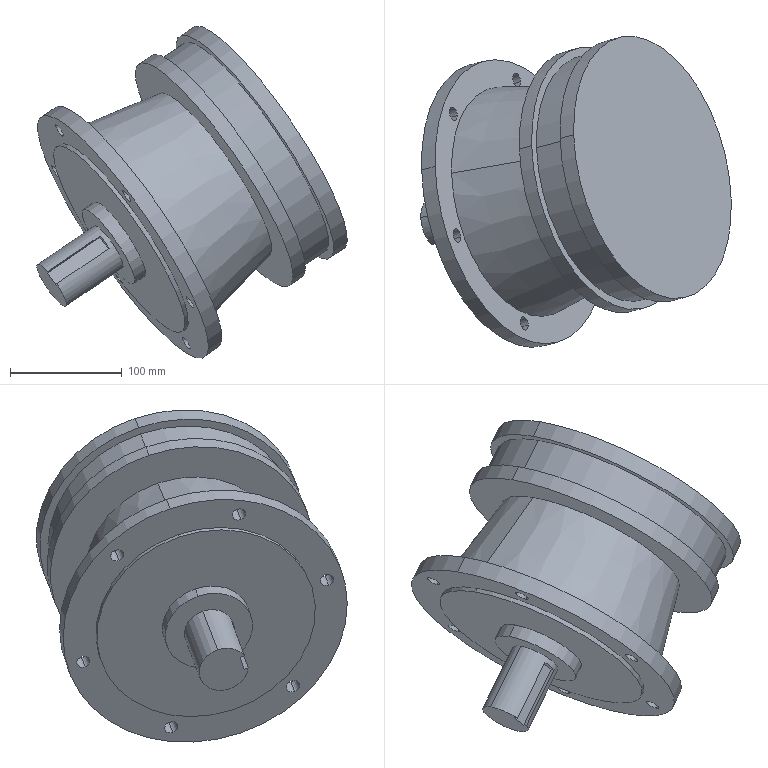Component | SolidWorks | XLD-4CycloidReducer-1 | 1 solid | 41 faces | box 277.92 x 278.17 x 297.34 mm | volume 6129226 mm3 | cylinder 26 | plane 13 | cone 2 | commonest cylinder face diameters 12.084 x12 240 x4 45 x2 80 x2 200 x2 260 x2 225.374 x2
build123d program:
from build123d import *

# Parameters (mm, degrees)
SKETCH2_R          = 40
EXTRUDE1_DEPTH     = 12
SKETCH3_R          = 22.5
EXTRUDE2_DEPTH     = 63
SKETCH4_W          = 14
SKETCH4_H          = 12.067
CUT_EXTRUDE1_DEPTH = 58
SKETCH5_R          = 6.042
CUT_EXTRUDE2_DEPTH = 40
CIRPATTERN1_COUNT  = 6


with BuildPart() as part:
    # Sketch1 → Revolve1 (revolve)
    with BuildSketch(Plane.XY, mode=Mode.PRIVATE) as revolve1_sk:
        Polygon((0, 0), (0, 100), (4, 100), (4, 130), (19, 130), (19, 105), (105, 87.671), (105, 120), (118.547, 120), (118.547, 112.687), (149.924, 112.687), (149.924, 120), (165, 120), (165, 0), align=None)
    revolve(revolve1_sk.sketch.rotate(Axis((0, 0, 0), (1, 0, 0)), 90), axis=Axis((0, 0, 0), (1, 0, 0)))

    # Sketch2 → Extrude1 (add)
    with BuildSketch(Plane.ZY):
        with Locations(Location((0, 0, 0), (0, 0, 180))):
            Circle(SKETCH2_R)
    extrude(amount=EXTRUDE1_DEPTH)

    # Sketch3 → Extrude2 (add)
    with BuildSketch(Plane.ZY.offset(12)):
        Circle(SKETCH3_R)
    extrude(amount=EXTRUDE2_DEPTH)

    # Sketch4 → Cut-Extrude1 (cut)
    with BuildSketch(Plane.ZY.offset(75)):
        with Locations((0, 23.534)):
            Rectangle(SKETCH4_W, SKETCH4_H)
    extrude(amount=-CUT_EXTRUDE1_DEPTH, mode=Mode.SUBTRACT)

    # Sketch5 → Cut-Extrude2 (cut)
    with BuildSketch(Plane.ZY.offset(-4)):
        with Locations((0, 115)):
            Circle(SKETCH5_R)
    cut_extrude2 = extrude(amount=-CUT_EXTRUDE2_DEPTH, mode=Mode.SUBTRACT)

    # CirPattern1: Cut-Extrude2 ×6 about axis
    cirpattern1_axis = Axis((0, 0, 0), (1, 0, 0))
    for i in range(1, CIRPATTERN1_COUNT):
        add(cut_extrude2.rotate(cirpattern1_axis, i * 360 / CIRPATTERN1_COUNT), mode=Mode.SUBTRACT)


solid = part.part

# Placed as in the assembly
solid = solid.moved(Location((474.122, -128.569, 107.181), (162.612, 35.968, -2.042)))